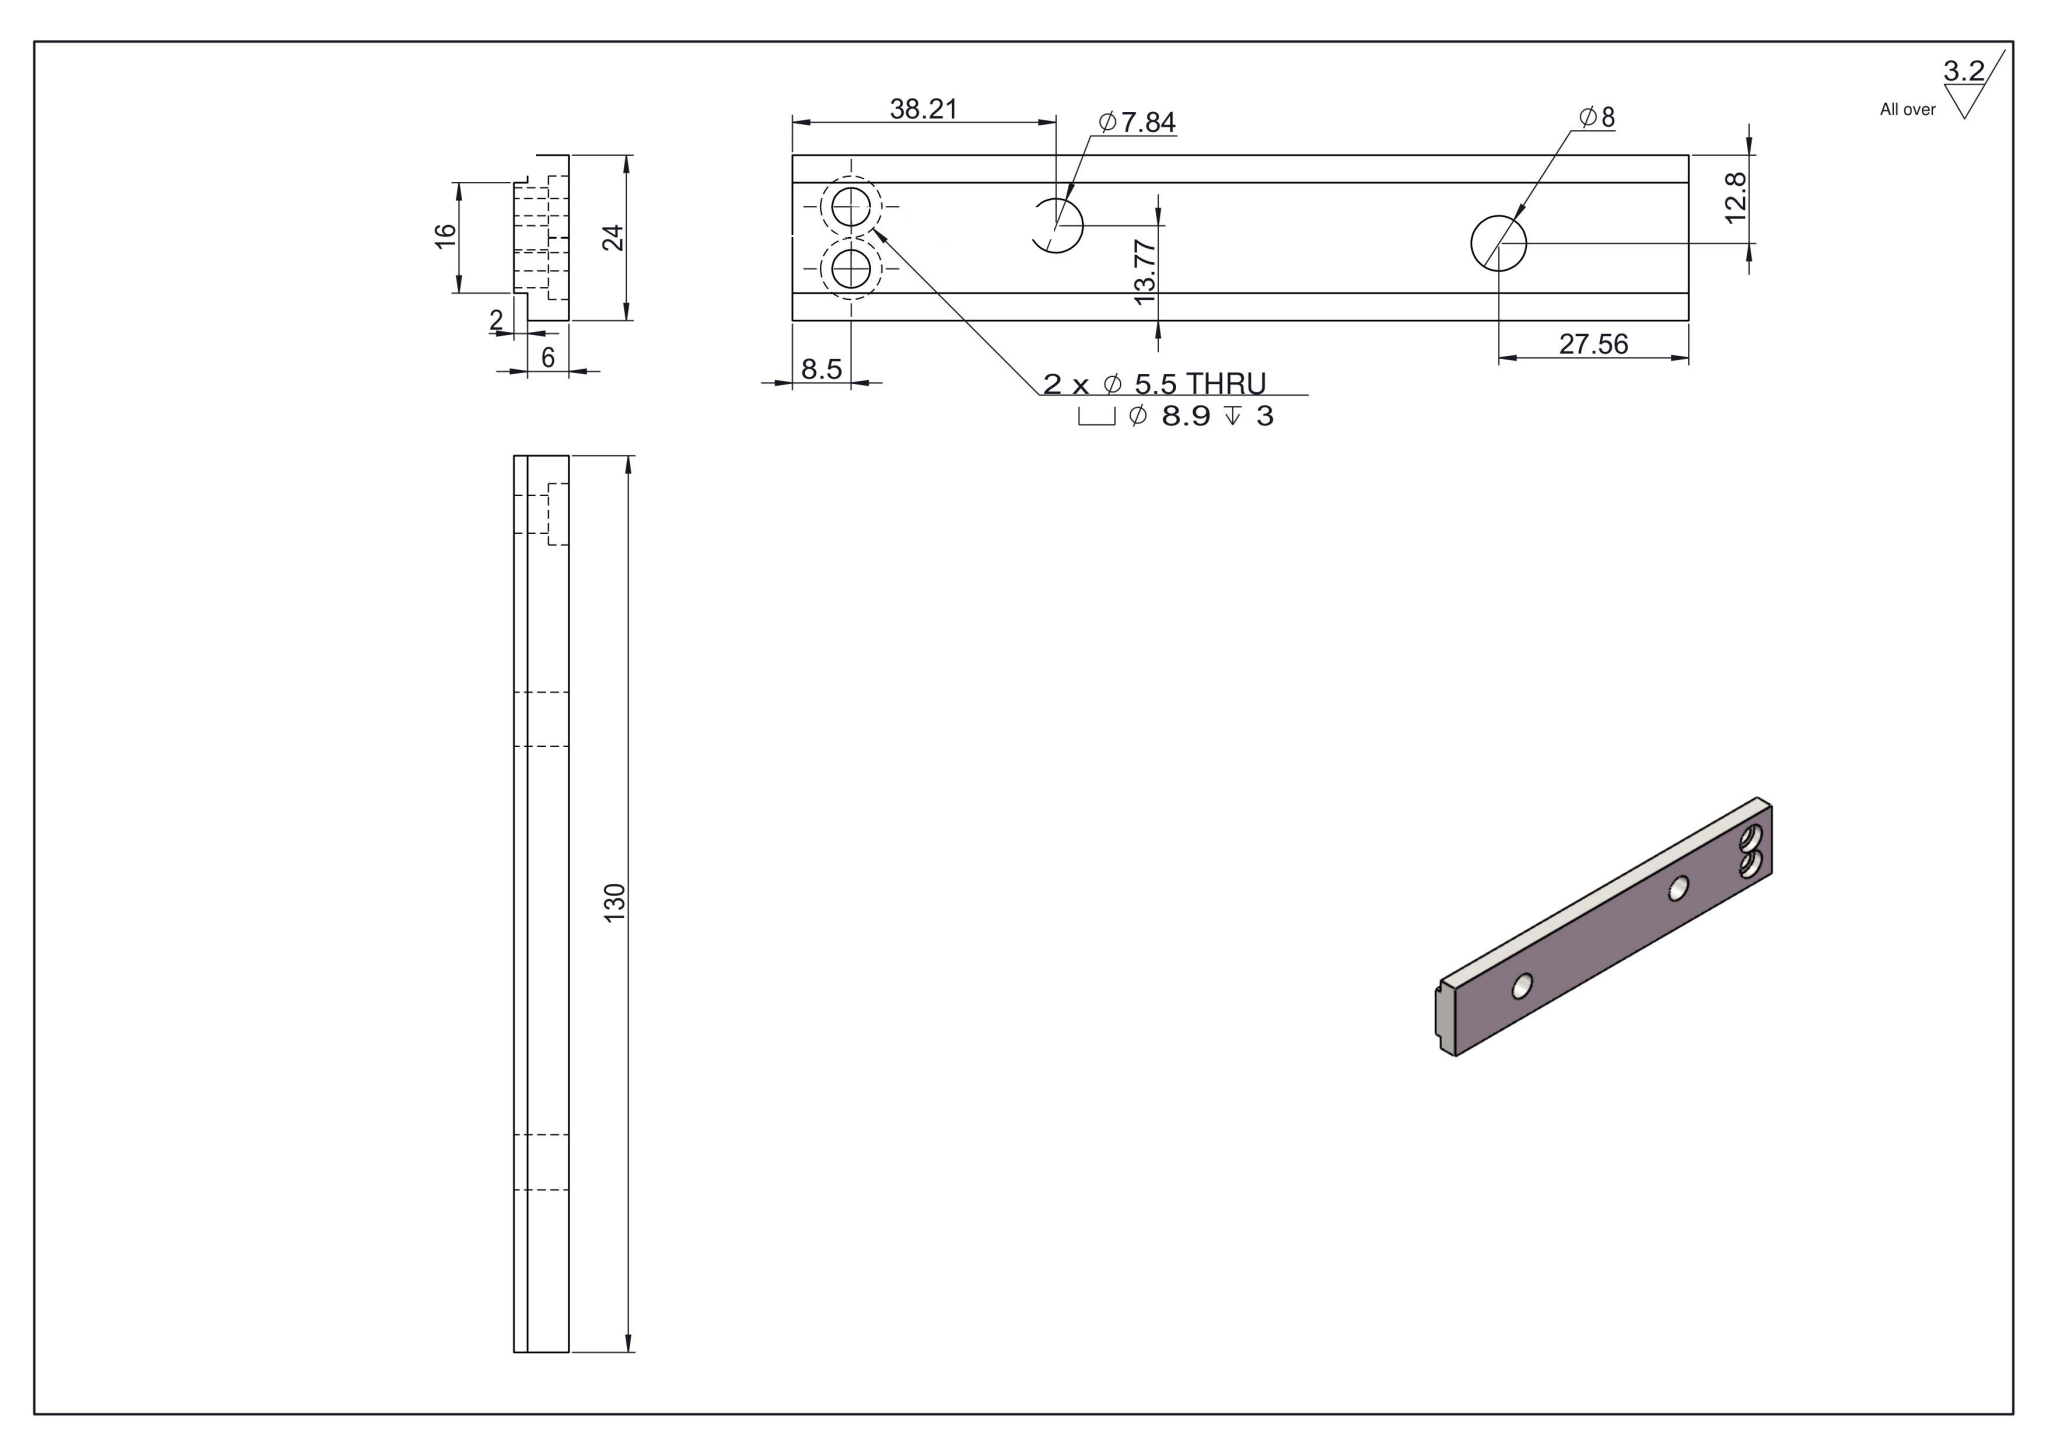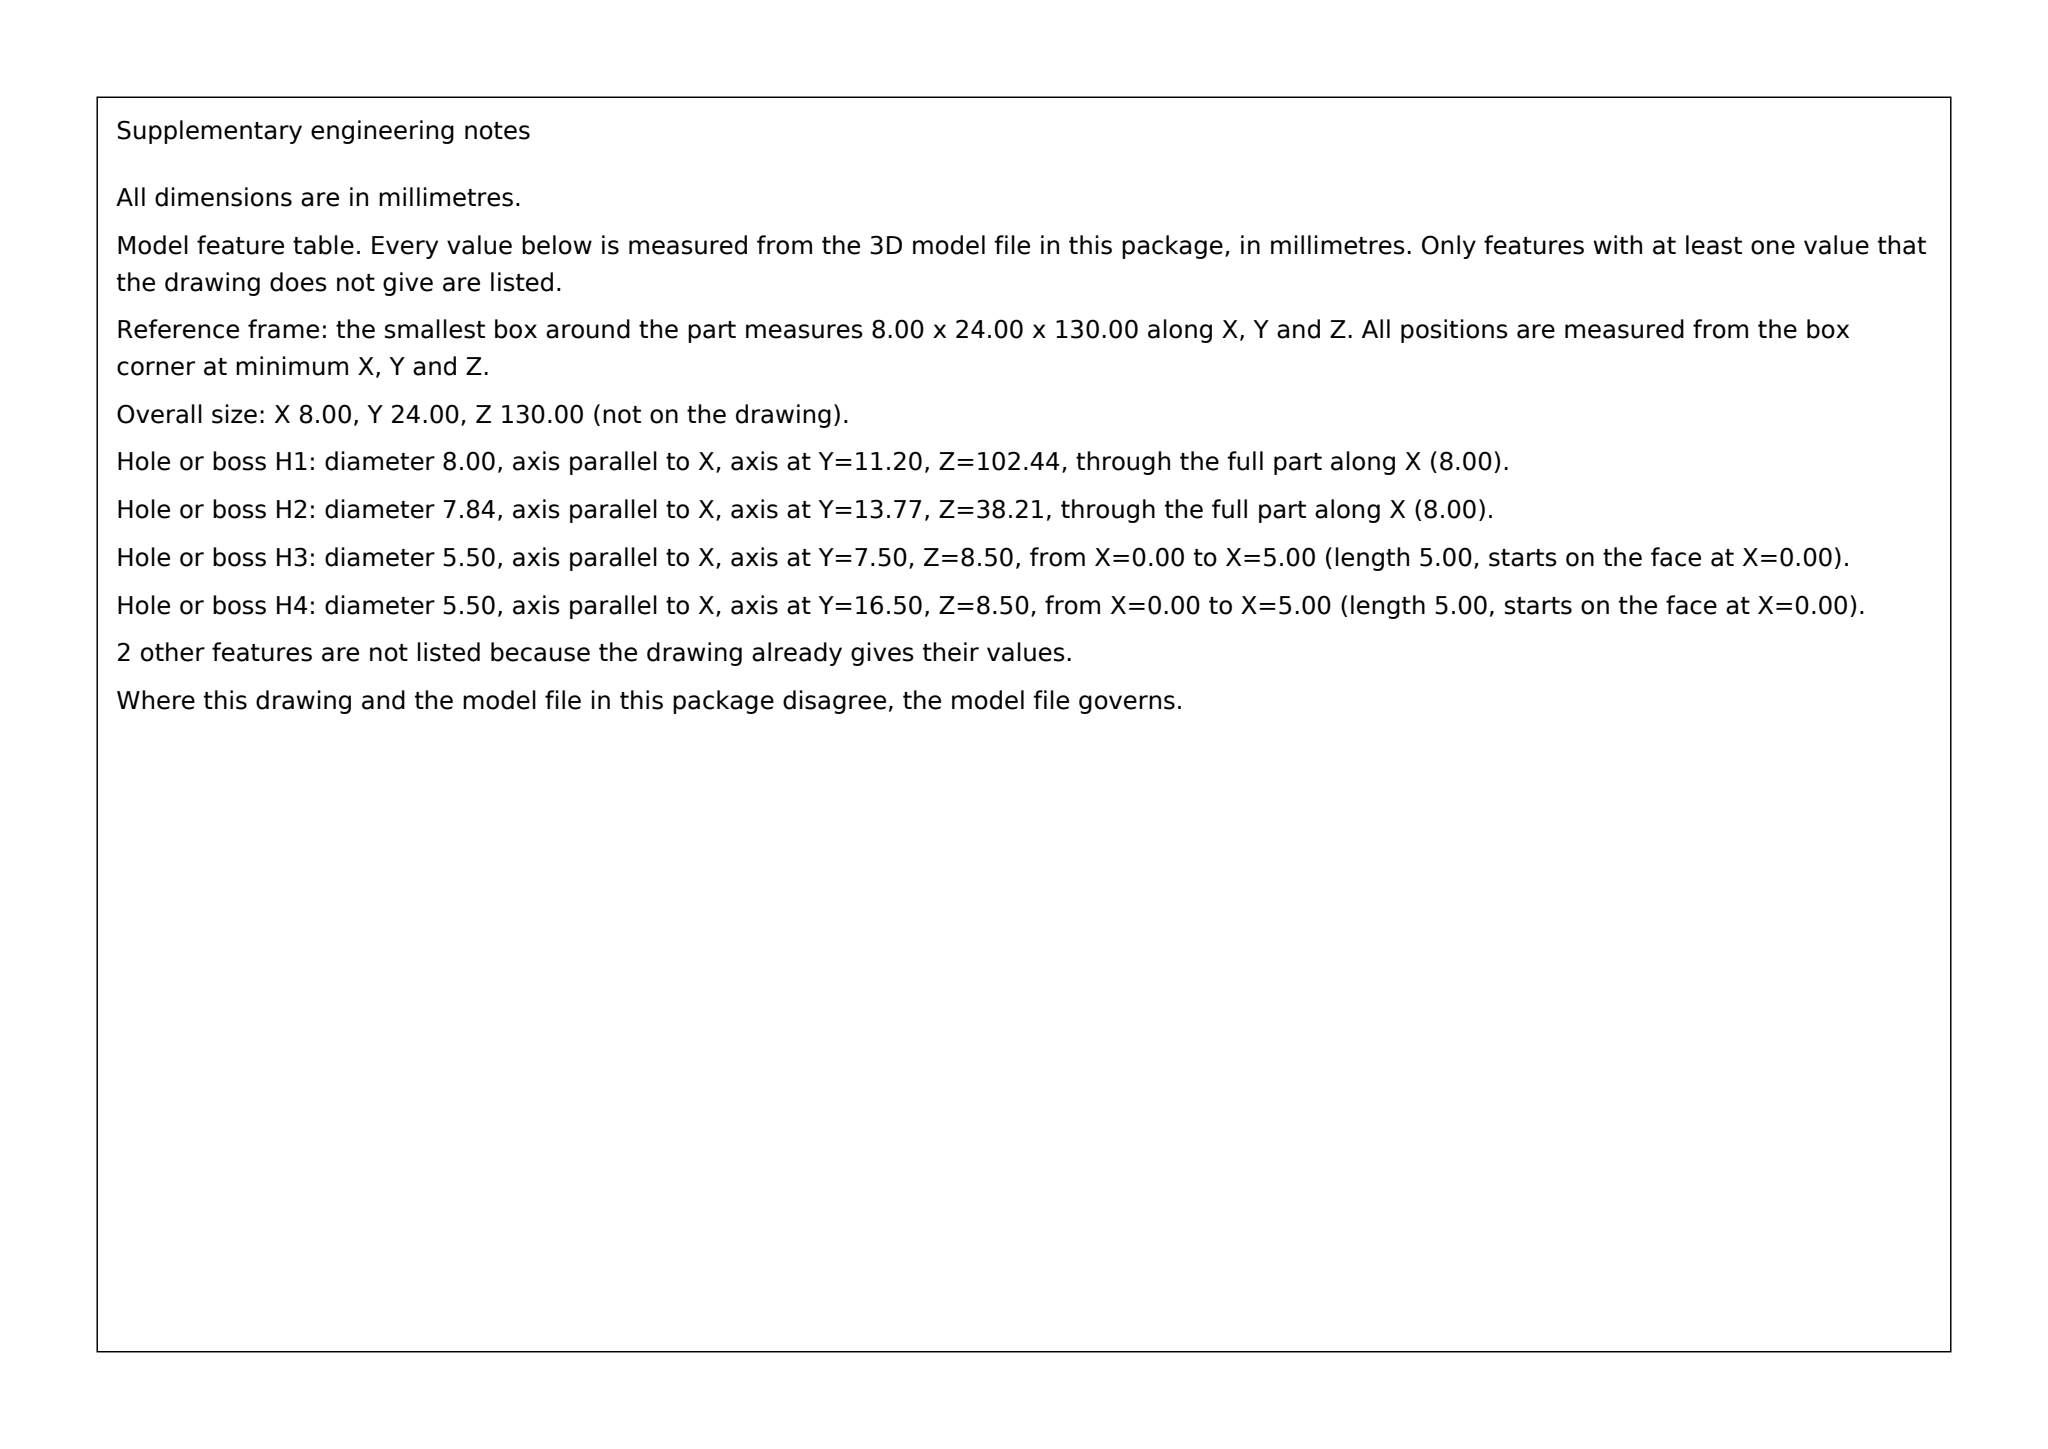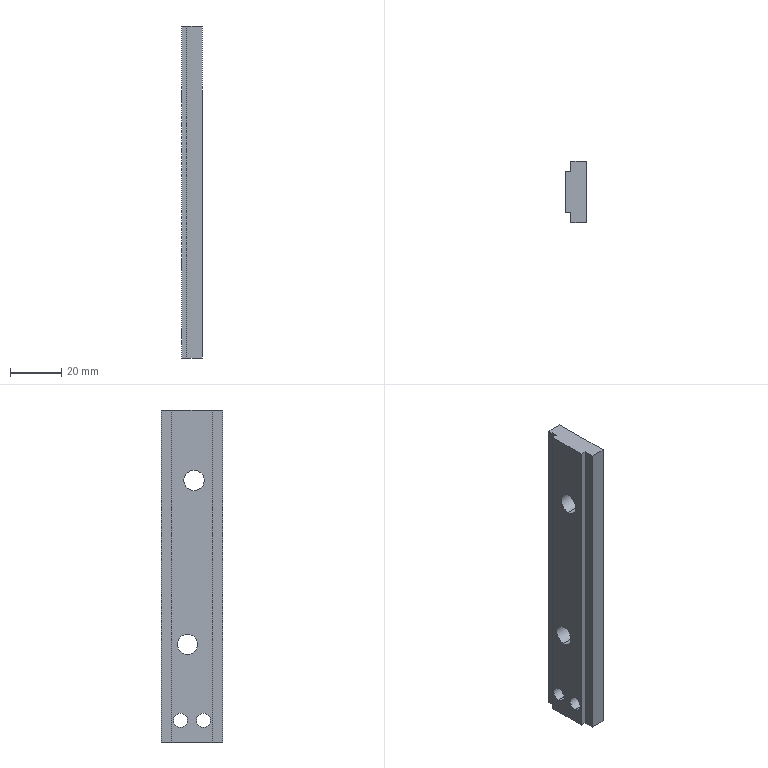Part | SolidWorks | mm | 1 solid | 24 faces | box 8 x 24 x 130 mm | volume 21481 mm3 | cylinder 12 | plane 12 | commonest cylinder face diameters 8.9 x4 5.5 x4 7.84 x2 7.997 x2
build123d program:
from build123d import *

# Parameters (mm, degrees)
BOSS_EXTRUDE1_DEPTH                             = 130
M5_HEX_SOCKET_HEAD_CAP_SCREW_CBORE2_D           = 5.5
M5_HEX_SOCKET_HEAD_CAP_SCREW_CBORE2_CBORE_D     = 8.9
M5_HEX_SOCKET_HEAD_CAP_SCREW_CBORE2_CBORE_DEPTH = 3
SKETCH4_R                                       = 3.92
SKETCH4_R_2                                     = 3.999
CUT_EXTRUDE1_DEPTH                              = 80


with BuildPart() as part:
    # Sketch1 → Boss-Extrude1 (new body)
    with BuildSketch(Plane.XY):
        Polygon((0, 0), (0, -16), (2, -16), (2, -20), (8, -20), (8, 4), (2, 4), (2, 0), align=None)
    extrude(amount=BOSS_EXTRUDE1_DEPTH)

    # M5 Hex Socket Head Cap Screw CBORE2 (through all)
    with Locations(Plane(origin=(8, 0, 0), x_dir=(0, 0, -1), z_dir=(1, 0, 0))):
        with Locations((-8.5, -3.5), (-8.5, -12.5)):
            CounterBoreHole(M5_HEX_SOCKET_HEAD_CAP_SCREW_CBORE2_D / 2, M5_HEX_SOCKET_HEAD_CAP_SCREW_CBORE2_CBORE_D / 2, M5_HEX_SOCKET_HEAD_CAP_SCREW_CBORE2_CBORE_DEPTH)

    # Sketch4 → Cut-Extrude1 (cut)
    with BuildSketch(Plane.ZY):
        with Locations((38.212, -6.229)):
            Circle(SKETCH4_R)
        with Locations((102.442, -8.805)):
            Circle(SKETCH4_R_2)
    extrude(amount=-CUT_EXTRUDE1_DEPTH, mode=Mode.SUBTRACT)


solid = part.part
STEP:
#1=CARTESIAN_POINT('',(8.,-6.229,34.292));
#2=VERTEX_POINT('',#1);
#3=CARTESIAN_POINT('',(8.,-6.229,42.132));
#4=VERTEX_POINT('',#3);
#5=CARTESIAN_POINT('',(8.,-6.229,38.212));
#6=DIRECTION('',(-1.,0.,0.));
#7=DIRECTION('',(0.,0.,1.));
#8=AXIS2_PLACEMENT_3D('',#5,#6,#7);
#9=CIRCLE('',#8,3.92);
#10=EDGE_CURVE('',#2,#4,#9,.T.);
#11=ORIENTED_EDGE('',*,*,#10,.F.);
#12=CARTESIAN_POINT('',(0.,-6.229,34.292));
#13=VERTEX_POINT('',#12);
#14=CARTESIAN_POINT('',(80.,-6.229,34.292));
#15=DIRECTION('',(-1.,0.,0.));
#16=VECTOR('',#15,1000.);
#17=LINE('',#14,#16);
#18=EDGE_CURVE('',#2,#13,#17,.T.);
#19=ORIENTED_EDGE('',*,*,#18,.T.);
#20=CARTESIAN_POINT('',(0.,-6.229,42.132));
#21=VERTEX_POINT('',#20);
#22=CARTESIAN_POINT('',(0.,-6.229,38.212));
#23=DIRECTION('',(-1.,0.,0.));
#24=DIRECTION('',(0.,0.,1.));
#25=AXIS2_PLACEMENT_3D('',#22,#23,#24);
#26=CIRCLE('',#25,3.92);
#27=EDGE_CURVE('',#13,#21,#26,.T.);
#28=ORIENTED_EDGE('',*,*,#27,.T.);
#29=CARTESIAN_POINT('',(80.,-6.229,42.132));
#30=DIRECTION('',(-1.,0.,0.));
#31=VECTOR('',#30,1000.);
#32=LINE('',#29,#31);
#33=EDGE_CURVE('',#4,#21,#32,.T.);
#34=ORIENTED_EDGE('',*,*,#33,.F.);
#35=EDGE_LOOP('',(#11,#19,#28,#34));
#36=FACE_OUTER_BOUND('',#35,.T.);
#37=CARTESIAN_POINT('',(80.,-6.229,38.212));
#38=DIRECTION('',(-1.,0.,0.));
#39=DIRECTION('',(0.,0.,1.));
#40=AXIS2_PLACEMENT_3D('',#37,#38,#39);
#41=CYLINDRICAL_SURFACE('',#40,3.92);
#42=ADVANCED_FACE('',(#36),#41,.F.);
#43=CARTESIAN_POINT('',(8.,-8.805,98.443));
#44=VERTEX_POINT('',#43);
#45=CARTESIAN_POINT('',(8.,-8.805,106.441));
#46=VERTEX_POINT('',#45);
#47=CARTESIAN_POINT('',(8.,-8.805,102.442));
#48=DIRECTION('',(-1.,0.,0.));
#49=DIRECTION('',(0.,0.,1.));
#50=AXIS2_PLACEMENT_3D('',#47,#48,#49);
#51=CIRCLE('',#50,3.999);
#52=EDGE_CURVE('',#44,#46,#51,.T.);
#53=ORIENTED_EDGE('',*,*,#52,.F.);
#54=CARTESIAN_POINT('',(0.,-8.805,98.443));
#55=VERTEX_POINT('',#54);
#56=CARTESIAN_POINT('',(80.,-8.805,98.443));
#57=DIRECTION('',(-1.,0.,0.));
#58=VECTOR('',#57,1000.);
#59=LINE('',#56,#58);
#60=EDGE_CURVE('',#44,#55,#59,.T.);
#61=ORIENTED_EDGE('',*,*,#60,.T.);
#62=CARTESIAN_POINT('',(0.,-8.805,106.441));
#63=VERTEX_POINT('',#62);
#64=CARTESIAN_POINT('',(0.,-8.805,102.442));
#65=DIRECTION('',(-1.,0.,0.));
#66=DIRECTION('',(0.,0.,1.));
#67=AXIS2_PLACEMENT_3D('',#64,#65,#66);
#68=CIRCLE('',#67,3.999);
#69=EDGE_CURVE('',#55,#63,#68,.T.);
#70=ORIENTED_EDGE('',*,*,#69,.T.);
#71=CARTESIAN_POINT('',(80.,-8.805,106.441));
#72=DIRECTION('',(-1.,0.,0.));
#73=VECTOR('',#72,1000.);
#74=LINE('',#71,#73);
#75=EDGE_CURVE('',#46,#63,#74,.T.);
#76=ORIENTED_EDGE('',*,*,#75,.F.);
#77=EDGE_LOOP('',(#53,#61,#70,#76));
#78=FACE_OUTER_BOUND('',#77,.T.);
#79=CARTESIAN_POINT('',(80.,-8.805,102.442));
#80=DIRECTION('',(-1.,0.,0.));
#81=DIRECTION('',(0.,0.,1.));
#82=AXIS2_PLACEMENT_3D('',#79,#80,#81);
#83=CYLINDRICAL_SURFACE('',#82,3.999);
#84=ADVANCED_FACE('',(#78),#83,.F.);
#85=CARTESIAN_POINT('',(5.,-3.5,12.95));
#86=VERTEX_POINT('',#85);
#87=CARTESIAN_POINT('',(5.,-3.5,4.05));
#88=VERTEX_POINT('',#87);
#89=CARTESIAN_POINT('',(5.,-3.5,8.5));
#90=DIRECTION('',(1.,0.,0.));
#91=DIRECTION('',(0.,0.,-1.));
#92=AXIS2_PLACEMENT_3D('',#89,#90,#91);
#93=CIRCLE('',#92,4.45);
#94=EDGE_CURVE('',#86,#88,#93,.T.);
#95=ORIENTED_EDGE('',*,*,#94,.F.);
#96=CARTESIAN_POINT('',(8.,-3.5,12.95));
#97=VERTEX_POINT('',#96);
#98=CARTESIAN_POINT('',(8.,-3.5,12.95));
#99=DIRECTION('',(1.,0.,0.));
#100=VECTOR('',#99,1000.);
#101=LINE('',#98,#100);
#102=EDGE_CURVE('',#86,#97,#101,.T.);
#103=ORIENTED_EDGE('',*,*,#102,.T.);
#104=CARTESIAN_POINT('',(8.,-3.5,4.05));
#105=VERTEX_POINT('',#104);
#106=CARTESIAN_POINT('',(8.,-3.5,8.5));
#107=DIRECTION('',(1.,0.,0.));
#108=DIRECTION('',(0.,0.,-1.));
#109=AXIS2_PLACEMENT_3D('',#106,#107,#108);
#110=CIRCLE('',#109,4.45);
#111=EDGE_CURVE('',#97,#105,#110,.T.);
#112=ORIENTED_EDGE('',*,*,#111,.T.);
#113=CARTESIAN_POINT('',(8.,-3.5,4.05));
#114=DIRECTION('',(1.,0.,0.));
#115=VECTOR('',#114,1000.);
#116=LINE('',#113,#115);
#117=EDGE_CURVE('',#88,#105,#116,.T.);
#118=ORIENTED_EDGE('',*,*,#117,.F.);
#119=EDGE_LOOP('',(#95,#103,#112,#118));
#120=FACE_OUTER_BOUND('',#119,.T.);
#121=CARTESIAN_POINT('',(8.,-3.5,8.5));
#122=DIRECTION('',(1.,0.,0.));
#123=DIRECTION('',(0.,0.,-1.));
#124=AXIS2_PLACEMENT_3D('',#121,#122,#123);
#125=CYLINDRICAL_SURFACE('',#124,4.45);
#126=ADVANCED_FACE('',(#120),#125,.F.);
#127=CARTESIAN_POINT('',(0.,-3.5,11.25));
#128=VERTEX_POINT('',#127);
#129=CARTESIAN_POINT('',(0.,-3.5,5.75));
#130=VERTEX_POINT('',#129);
#131=CARTESIAN_POINT('',(0.,-3.5,8.5));
#132=DIRECTION('',(1.,0.,0.));
#133=DIRECTION('',(0.,0.,-1.));
#134=AXIS2_PLACEMENT_3D('',#131,#132,#133);
#135=CIRCLE('',#134,2.75);
#136=EDGE_CURVE('',#128,#130,#135,.T.);
#137=ORIENTED_EDGE('',*,*,#136,.F.);
#138=CARTESIAN_POINT('',(5.,-3.5,11.25));
#139=VERTEX_POINT('',#138);
#140=CARTESIAN_POINT('',(8.,-3.5,11.25));
#141=DIRECTION('',(1.,0.,0.));
#142=VECTOR('',#141,1000.);
#143=LINE('',#140,#142);
#144=EDGE_CURVE('',#128,#139,#143,.T.);
#145=ORIENTED_EDGE('',*,*,#144,.T.);
#146=CARTESIAN_POINT('',(5.,-3.5,5.75));
#147=VERTEX_POINT('',#146);
#148=CARTESIAN_POINT('',(5.,-3.5,8.5));
#149=DIRECTION('',(1.,0.,0.));
#150=DIRECTION('',(0.,0.,-1.));
#151=AXIS2_PLACEMENT_3D('',#148,#149,#150);
#152=CIRCLE('',#151,2.75);
#153=EDGE_CURVE('',#139,#147,#152,.T.);
#154=ORIENTED_EDGE('',*,*,#153,.T.);
#155=CARTESIAN_POINT('',(8.,-3.5,5.75));
#156=DIRECTION('',(1.,0.,0.));
#157=VECTOR('',#156,1000.);
#158=LINE('',#155,#157);
#159=EDGE_CURVE('',#130,#147,#158,.T.);
#160=ORIENTED_EDGE('',*,*,#159,.F.);
#161=EDGE_LOOP('',(#137,#145,#154,#160));
#162=FACE_OUTER_BOUND('',#161,.T.);
#163=CARTESIAN_POINT('',(8.,-3.5,8.5));
#164=DIRECTION('',(1.,0.,0.));
#165=DIRECTION('',(0.,0.,-1.));
#166=AXIS2_PLACEMENT_3D('',#163,#164,#165);
#167=CYLINDRICAL_SURFACE('',#166,2.75);
#168=ADVANCED_FACE('',(#162),#167,.F.);
#169=CARTESIAN_POINT('',(5.,-12.5,12.95));
#170=VERTEX_POINT('',#169);
#171=CARTESIAN_POINT('',(5.,-12.5,4.05));
#172=VERTEX_POINT('',#171);
#173=CARTESIAN_POINT('',(5.,-12.5,8.5));
#174=DIRECTION('',(1.,0.,0.));
#175=DIRECTION('',(0.,0.,-1.));
#176=AXIS2_PLACEMENT_3D('',#173,#174,#175);
#177=CIRCLE('',#176,4.45);
#178=EDGE_CURVE('',#170,#172,#177,.T.);
#179=ORIENTED_EDGE('',*,*,#178,.F.);
#180=CARTESIAN_POINT('',(8.,-12.5,12.95));
#181=VERTEX_POINT('',#180);
#182=CARTESIAN_POINT('',(8.,-12.5,12.95));
#183=DIRECTION('',(1.,0.,0.));
#184=VECTOR('',#183,1000.);
#185=LINE('',#182,#184);
#186=EDGE_CURVE('',#170,#181,#185,.T.);
#187=ORIENTED_EDGE('',*,*,#186,.T.);
#188=CARTESIAN_POINT('',(8.,-12.5,4.05));
#189=VERTEX_POINT('',#188);
#190=CARTESIAN_POINT('',(8.,-12.5,8.5));
#191=DIRECTION('',(1.,0.,0.));
#192=DIRECTION('',(0.,0.,-1.));
#193=AXIS2_PLACEMENT_3D('',#190,#191,#192);
#194=CIRCLE('',#193,4.45);
#195=EDGE_CURVE('',#181,#189,#194,.T.);
#196=ORIENTED_EDGE('',*,*,#195,.T.);
#197=CARTESIAN_POINT('',(8.,-12.5,4.05));
#198=DIRECTION('',(1.,0.,0.));
#199=VECTOR('',#198,1000.);
#200=LINE('',#197,#199);
#201=EDGE_CURVE('',#172,#189,#200,.T.);
#202=ORIENTED_EDGE('',*,*,#201,.F.);
#203=EDGE_LOOP('',(#179,#187,#196,#202));
#204=FACE_OUTER_BOUND('',#203,.T.);
#205=CARTESIAN_POINT('',(8.,-12.5,8.5));
#206=DIRECTION('',(1.,0.,0.));
#207=DIRECTION('',(0.,0.,-1.));
#208=AXIS2_PLACEMENT_3D('',#205,#206,#207);
#209=CYLINDRICAL_SURFACE('',#208,4.45);
#210=ADVANCED_FACE('',(#204),#209,.F.);
#211=CARTESIAN_POINT('',(0.,-12.5,11.25));
#212=VERTEX_POINT('',#211);
#213=CARTESIAN_POINT('',(0.,-12.5,5.75));
#214=VERTEX_POINT('',#213);
#215=CARTESIAN_POINT('',(0.,-12.5,8.5));
#216=DIRECTION('',(1.,0.,0.));
#217=DIRECTION('',(0.,0.,-1.));
#218=AXIS2_PLACEMENT_3D('',#215,#216,#217);
#219=CIRCLE('',#218,2.75);
#220=EDGE_CURVE('',#212,#214,#219,.T.);
#221=ORIENTED_EDGE('',*,*,#220,.F.);
#222=CARTESIAN_POINT('',(5.,-12.5,11.25));
#223=VERTEX_POINT('',#222);
#224=CARTESIAN_POINT('',(8.,-12.5,11.25));
#225=DIRECTION('',(1.,0.,0.));
#226=VECTOR('',#225,1000.);
#227=LINE('',#224,#226);
#228=EDGE_CURVE('',#212,#223,#227,.T.);
#229=ORIENTED_EDGE('',*,*,#228,.T.);
#230=CARTESIAN_POINT('',(5.,-12.5,5.75));
#231=VERTEX_POINT('',#230);
#232=CARTESIAN_POINT('',(5.,-12.5,8.5));
#233=DIRECTION('',(1.,0.,0.));
#234=DIRECTION('',(0.,0.,-1.));
#235=AXIS2_PLACEMENT_3D('',#232,#233,#234);
#236=CIRCLE('',#235,2.75);
#237=EDGE_CURVE('',#223,#231,#236,.T.);
#238=ORIENTED_EDGE('',*,*,#237,.T.);
#239=CARTESIAN_POINT('',(8.,-12.5,5.75));
#240=DIRECTION('',(1.,0.,0.));
#241=VECTOR('',#240,1000.);
#242=LINE('',#239,#241);
#243=EDGE_CURVE('',#214,#231,#242,.T.);
#244=ORIENTED_EDGE('',*,*,#243,.F.);
#245=EDGE_LOOP('',(#221,#229,#238,#244));
#246=FACE_OUTER_BOUND('',#245,.T.);
#247=CARTESIAN_POINT('',(8.,-12.5,8.5));
#248=DIRECTION('',(1.,0.,0.));
#249=DIRECTION('',(0.,0.,-1.));
#250=AXIS2_PLACEMENT_3D('',#247,#248,#249);
#251=CYLINDRICAL_SURFACE('',#250,2.75);
#252=ADVANCED_FACE('',(#246),#251,.F.);
#253=CARTESIAN_POINT('',(8.,-6.229,38.212));
#254=DIRECTION('',(-1.,0.,0.));
#255=DIRECTION('',(0.,0.,1.));
#256=AXIS2_PLACEMENT_3D('',#253,#254,#255);
#257=CIRCLE('',#256,3.92);
#258=EDGE_CURVE('',#4,#2,#257,.T.);
#259=ORIENTED_EDGE('',*,*,#258,.T.);
#260=ORIENTED_EDGE('',*,*,#10,.T.);
#261=EDGE_LOOP('',(#259,#260));
#262=FACE_BOUND('',#261,.T.);
#263=CARTESIAN_POINT('',(8.,-8.805,102.442));
#264=DIRECTION('',(-1.,0.,0.));
#265=DIRECTION('',(0.,0.,1.));
#266=AXIS2_PLACEMENT_3D('',#263,#264,#265);
#267=CIRCLE('',#266,3.999);
#268=EDGE_CURVE('',#46,#44,#267,.T.);
#269=ORIENTED_EDGE('',*,*,#268,.T.);
#270=ORIENTED_EDGE('',*,*,#52,.T.);
#271=EDGE_LOOP('',(#269,#270));
#272=FACE_BOUND('',#271,.T.);
#273=CARTESIAN_POINT('',(8.,-12.5,8.5));
#274=DIRECTION('',(1.,0.,0.));
#275=DIRECTION('',(0.,0.,-1.));
#276=AXIS2_PLACEMENT_3D('',#273,#274,#275);
#277=CIRCLE('',#276,4.45);
#278=EDGE_CURVE('',#189,#181,#277,.T.);
#279=ORIENTED_EDGE('',*,*,#278,.F.);
#280=ORIENTED_EDGE('',*,*,#195,.F.);
#281=EDGE_LOOP('',(#279,#280));
#282=FACE_BOUND('',#281,.T.);
#283=CARTESIAN_POINT('',(8.,-20.,0.));
#284=VERTEX_POINT('',#283);
#285=CARTESIAN_POINT('',(8.,4.,0.));
#286=VERTEX_POINT('',#285);
#287=CARTESIAN_POINT('',(8.,-20.,0.));
#288=DIRECTION('',(0.,1.,0.));
#289=VECTOR('',#288,1000.);
#290=LINE('',#287,#289);
#291=EDGE_CURVE('',#284,#286,#290,.T.);
#292=ORIENTED_EDGE('',*,*,#291,.T.);
#293=CARTESIAN_POINT('',(8.,4.,130.));
#294=VERTEX_POINT('',#293);
#295=CARTESIAN_POINT('',(8.,4.,130.));
#296=DIRECTION('',(0.,0.,-1.));
#297=VECTOR('',#296,1000.);
#298=LINE('',#295,#297);
#299=EDGE_CURVE('',#294,#286,#298,.T.);
#300=ORIENTED_EDGE('',*,*,#299,.F.);
#301=CARTESIAN_POINT('',(8.,-20.,130.));
#302=VERTEX_POINT('',#301);
#303=CARTESIAN_POINT('',(8.,-20.,130.));
#304=DIRECTION('',(0.,1.,0.));
#305=VECTOR('',#304,1000.);
#306=LINE('',#303,#305);
#307=EDGE_CURVE('',#302,#294,#306,.T.);
#308=ORIENTED_EDGE('',*,*,#307,.F.);
#309=CARTESIAN_POINT('',(8.,-20.,130.));
#310=DIRECTION('',(0.,0.,-1.));
#311=VECTOR('',#310,1000.);
#312=LINE('',#309,#311);
#313=EDGE_CURVE('',#302,#284,#312,.T.);
#314=ORIENTED_EDGE('',*,*,#313,.T.);
#315=EDGE_LOOP('',(#292,#300,#308,#314));
#316=FACE_OUTER_BOUND('',#315,.T.);
#317=CARTESIAN_POINT('',(8.,-3.5,8.5));
#318=DIRECTION('',(1.,0.,0.));
#319=DIRECTION('',(0.,0.,-1.));
#320=AXIS2_PLACEMENT_3D('',#317,#318,#319);
#321=CIRCLE('',#320,4.45);
#322=EDGE_CURVE('',#105,#97,#321,.T.);
#323=ORIENTED_EDGE('',*,*,#322,.F.);
#324=ORIENTED_EDGE('',*,*,#111,.F.);
#325=EDGE_LOOP('',(#323,#324));
#326=FACE_BOUND('',#325,.T.);
#327=CARTESIAN_POINT('',(8.,-20.,130.));
#328=DIRECTION('',(-1.,0.,0.));
#329=DIRECTION('',(0.,0.,1.));
#330=AXIS2_PLACEMENT_3D('',#327,#328,#329);
#331=PLANE('',#330);
#332=ADVANCED_FACE('',(#262,#272,#282,#316,#326),#331,.F.);
#333=CARTESIAN_POINT('',(2.,-0.,0.));
#334=VERTEX_POINT('',#333);
#335=CARTESIAN_POINT('',(0.,0.,0.));
#336=VERTEX_POINT('',#335);
#337=CARTESIAN_POINT('',(2.,-0.,0.));
#338=DIRECTION('',(-1.,0.,0.));
#339=VECTOR('',#338,1000.);
#340=LINE('',#337,#339);
#341=EDGE_CURVE('',#334,#336,#340,.T.);
#342=ORIENTED_EDGE('',*,*,#341,.T.);
#343=CARTESIAN_POINT('',(0.,0.,130.));
#344=VERTEX_POINT('',#343);
#345=CARTESIAN_POINT('',(0.,0.,130.));
#346=DIRECTION('',(0.,0.,-1.));
#347=VECTOR('',#346,1000.);
#348=LINE('',#345,#347);
#349=EDGE_CURVE('',#344,#336,#348,.T.);
#350=ORIENTED_EDGE('',*,*,#349,.F.);
#351=CARTESIAN_POINT('',(2.,-0.,130.));
#352=VERTEX_POINT('',#351);
#353=CARTESIAN_POINT('',(2.,-0.,130.));
#354=DIRECTION('',(-1.,0.,0.));
#355=VECTOR('',#354,1000.);
#356=LINE('',#353,#355);
#357=EDGE_CURVE('',#352,#344,#356,.T.);
#358=ORIENTED_EDGE('',*,*,#357,.F.);
#359=CARTESIAN_POINT('',(2.,-0.,130.));
#360=DIRECTION('',(0.,0.,-1.));
#361=VECTOR('',#360,1000.);
#362=LINE('',#359,#361);
#363=EDGE_CURVE('',#352,#334,#362,.T.);
#364=ORIENTED_EDGE('',*,*,#363,.T.);
#365=EDGE_LOOP('',(#342,#350,#358,#364));
#366=FACE_OUTER_BOUND('',#365,.T.);
#367=CARTESIAN_POINT('',(2.,-0.,130.));
#368=DIRECTION('',(-0.,-1.,0.));
#369=DIRECTION('',(1.,-0.,0.));
#370=AXIS2_PLACEMENT_3D('',#367,#368,#369);
#371=PLANE('',#370);
#372=ADVANCED_FACE('',(#366),#371,.F.);
#373=CARTESIAN_POINT('',(0.,-6.229,38.212));
#374=DIRECTION('',(-1.,0.,0.));
#375=DIRECTION('',(0.,0.,1.));
#376=AXIS2_PLACEMENT_3D('',#373,#374,#375);
#377=CIRCLE('',#376,3.92);
#378=EDGE_CURVE('',#21,#13,#377,.T.);
#379=ORIENTED_EDGE('',*,*,#378,.F.);
#380=ORIENTED_EDGE('',*,*,#27,.F.);
#381=EDGE_LOOP('',(#379,#380));
#382=FACE_BOUND('',#381,.T.);
#383=CARTESIAN_POINT('',(0.,-8.805,102.442));
#384=DIRECTION('',(-1.,0.,0.));
#385=DIRECTION('',(0.,0.,1.));
#386=AXIS2_PLACEMENT_3D('',#383,#384,#385);
#387=CIRCLE('',#386,3.999);
#388=EDGE_CURVE('',#63,#55,#387,.T.);
#389=ORIENTED_EDGE('',*,*,#388,.F.);
#390=ORIENTED_EDGE('',*,*,#69,.F.);
#391=EDGE_LOOP('',(#389,#390));
#392=FACE_BOUND('',#391,.T.);
#393=CARTESIAN_POINT('',(0.,-3.5,8.5));
#394=DIRECTION('',(1.,0.,0.));
#395=DIRECTION('',(0.,0.,-1.));
#396=AXIS2_PLACEMENT_3D('',#393,#394,#395);
#397=CIRCLE('',#396,2.75);
#398=EDGE_CURVE('',#130,#128,#397,.T.);
#399=ORIENTED_EDGE('',*,*,#398,.T.);
#400=ORIENTED_EDGE('',*,*,#136,.T.);
#401=EDGE_LOOP('',(#399,#400));
#402=FACE_BOUND('',#401,.T.);
#403=CARTESIAN_POINT('',(0.,-12.5,8.5));
#404=DIRECTION('',(1.,0.,0.));
#405=DIRECTION('',(0.,0.,-1.));
#406=AXIS2_PLACEMENT_3D('',#403,#404,#405);
#407=CIRCLE('',#406,2.75);
#408=EDGE_CURVE('',#214,#212,#407,.T.);
#409=ORIENTED_EDGE('',*,*,#408,.T.);
#410=ORIENTED_EDGE('',*,*,#220,.T.);
#411=EDGE_LOOP('',(#409,#410));
#412=FACE_BOUND('',#411,.T.);
#413=CARTESIAN_POINT('',(0.,-16.,0.));
#414=VERTEX_POINT('',#413);
#415=CARTESIAN_POINT('',(0.,0.,0.));
#416=DIRECTION('',(0.,-1.,0.));
#417=VECTOR('',#416,1000.);
#418=LINE('',#415,#417);
#419=EDGE_CURVE('',#336,#414,#418,.T.);
#420=ORIENTED_EDGE('',*,*,#419,.T.);
#421=CARTESIAN_POINT('',(0.,-16.,130.));
#422=VERTEX_POINT('',#421);
#423=CARTESIAN_POINT('',(0.,-16.,130.));
#424=DIRECTION('',(0.,0.,-1.));
#425=VECTOR('',#424,1000.);
#426=LINE('',#423,#425);
#427=EDGE_CURVE('',#422,#414,#426,.T.);
#428=ORIENTED_EDGE('',*,*,#427,.F.);
#429=CARTESIAN_POINT('',(0.,0.,130.));
#430=DIRECTION('',(0.,-1.,0.));
#431=VECTOR('',#430,1000.);
#432=LINE('',#429,#431);
#433=EDGE_CURVE('',#344,#422,#432,.T.);
#434=ORIENTED_EDGE('',*,*,#433,.F.);
#435=ORIENTED_EDGE('',*,*,#349,.T.);
#436=EDGE_LOOP('',(#420,#428,#434,#435));
#437=FACE_OUTER_BOUND('',#436,.T.);
#438=CARTESIAN_POINT('',(0.,0.,130.));
#439=DIRECTION('',(1.,0.,0.));
#440=DIRECTION('',(0.,0.,-1.));
#441=AXIS2_PLACEMENT_3D('',#438,#439,#440);
#442=PLANE('',#441);
#443=ADVANCED_FACE('',(#382,#392,#402,#412,#437),#442,.F.);
#444=CARTESIAN_POINT('',(2.,-16.,0.));
#445=VERTEX_POINT('',#444);
#446=CARTESIAN_POINT('',(0.,-16.,0.));
#447=DIRECTION('',(1.,0.,0.));
#448=VECTOR('',#447,1000.);
#449=LINE('',#446,#448);
#450=EDGE_CURVE('',#414,#445,#449,.T.);
#451=ORIENTED_EDGE('',*,*,#450,.T.);
#452=CARTESIAN_POINT('',(2.,-16.,130.));
#453=VERTEX_POINT('',#452);
#454=CARTESIAN_POINT('',(2.,-16.,130.));
#455=DIRECTION('',(0.,0.,-1.));
#456=VECTOR('',#455,1000.);
#457=LINE('',#454,#456);
#458=EDGE_CURVE('',#453,#445,#457,.T.);
#459=ORIENTED_EDGE('',*,*,#458,.F.);
#460=CARTESIAN_POINT('',(0.,-16.,130.));
#461=DIRECTION('',(1.,0.,0.));
#462=VECTOR('',#461,1000.);
#463=LINE('',#460,#462);
#464=EDGE_CURVE('',#422,#453,#463,.T.);
#465=ORIENTED_EDGE('',*,*,#464,.F.);
#466=ORIENTED_EDGE('',*,*,#427,.T.);
#467=EDGE_LOOP('',(#451,#459,#465,#466));
#468=FACE_OUTER_BOUND('',#467,.T.);
#469=CARTESIAN_POINT('',(0.,-16.,130.));
#470=DIRECTION('',(0.,1.,0.));
#471=DIRECTION('',(0.,0.,1.));
#472=AXIS2_PLACEMENT_3D('',#469,#470,#471);
#473=PLANE('',#472);
#474=ADVANCED_FACE('',(#468),#473,.F.);
#475=CARTESIAN_POINT('',(2.,-20.,0.));
#476=VERTEX_POINT('',#475);
#477=CARTESIAN_POINT('',(2.,-16.,0.));
#478=DIRECTION('',(0.,-1.,0.));
#479=VECTOR('',#478,1000.);
#480=LINE('',#477,#479);
#481=EDGE_CURVE('',#445,#476,#480,.T.);
#482=ORIENTED_EDGE('',*,*,#481,.T.);
#483=CARTESIAN_POINT('',(2.,-20.,130.));
#484=VERTEX_POINT('',#483);
#485=CARTESIAN_POINT('',(2.,-20.,130.));
#486=DIRECTION('',(0.,0.,-1.));
#487=VECTOR('',#486,1000.);
#488=LINE('',#485,#487);
#489=EDGE_CURVE('',#484,#476,#488,.T.);
#490=ORIENTED_EDGE('',*,*,#489,.F.);
#491=CARTESIAN_POINT('',(2.,-16.,130.));
#492=DIRECTION('',(0.,-1.,0.));
#493=VECTOR('',#492,1000.);
#494=LINE('',#491,#493);
#495=EDGE_CURVE('',#453,#484,#494,.T.);
#496=ORIENTED_EDGE('',*,*,#495,.F.);
#497=ORIENTED_EDGE('',*,*,#458,.T.);
#498=EDGE_LOOP('',(#482,#490,#496,#497));
#499=FACE_OUTER_BOUND('',#498,.T.);
#500=CARTESIAN_POINT('',(2.,-16.,130.));
#501=DIRECTION('',(1.,0.,0.));
#502=DIRECTION('',(0.,0.,-1.));
#503=AXIS2_PLACEMENT_3D('',#500,#501,#502);
#504=PLANE('',#503);
#505=ADVANCED_FACE('',(#499),#504,.F.);
#506=CARTESIAN_POINT('',(2.,-20.,0.));
#507=DIRECTION('',(1.,0.,0.));
#508=VECTOR('',#507,1000.);
#509=LINE('',#506,#508);
#510=EDGE_CURVE('',#476,#284,#509,.T.);
#511=ORIENTED_EDGE('',*,*,#510,.T.);
#512=ORIENTED_EDGE('',*,*,#313,.F.);
#513=CARTESIAN_POINT('',(2.,-20.,130.));
#514=DIRECTION('',(1.,0.,0.));
#515=VECTOR('',#514,1000.);
#516=LINE('',#513,#515);
#517=EDGE_CURVE('',#484,#302,#516,.T.);
#518=ORIENTED_EDGE('',*,*,#517,.F.);
#519=ORIENTED_EDGE('',*,*,#489,.T.);
#520=EDGE_LOOP('',(#511,#512,#518,#519));
#521=FACE_OUTER_BOUND('',#520,.T.);
#522=CARTESIAN_POINT('',(2.,-20.,130.));
#523=DIRECTION('',(0.,1.,0.));
#524=DIRECTION('',(0.,0.,1.));
#525=AXIS2_PLACEMENT_3D('',#522,#523,#524);
#526=PLANE('',#525);
#527=ADVANCED_FACE('',(#521),#526,.F.);
#528=CARTESIAN_POINT('',(2.,4.,0.));
#529=VERTEX_POINT('',#528);
#530=CARTESIAN_POINT('',(8.,4.,0.));
#531=DIRECTION('',(-1.,0.,0.));
#532=VECTOR('',#531,1000.);
#533=LINE('',#530,#532);
#534=EDGE_CURVE('',#286,#529,#533,.T.);
#535=ORIENTED_EDGE('',*,*,#534,.T.);
#536=CARTESIAN_POINT('',(2.,4.,130.));
#537=VERTEX_POINT('',#536);
#538=CARTESIAN_POINT('',(2.,4.,130.));
#539=DIRECTION('',(0.,0.,-1.));
#540=VECTOR('',#539,1000.);
#541=LINE('',#538,#540);
#542=EDGE_CURVE('',#537,#529,#541,.T.);
#543=ORIENTED_EDGE('',*,*,#542,.F.);
#544=CARTESIAN_POINT('',(8.,4.,130.));
#545=DIRECTION('',(-1.,0.,0.));
#546=VECTOR('',#545,1000.);
#547=LINE('',#544,#546);
#548=EDGE_CURVE('',#294,#537,#547,.T.);
#549=ORIENTED_EDGE('',*,*,#548,.F.);
#550=ORIENTED_EDGE('',*,*,#299,.T.);
#551=EDGE_LOOP('',(#535,#543,#549,#550));
#552=FACE_OUTER_BOUND('',#551,.T.);
#553=CARTESIAN_POINT('',(8.,4.,130.));
#554=DIRECTION('',(0.,-1.,0.));
#555=DIRECTION('',(0.,0.,-1.));
#556=AXIS2_PLACEMENT_3D('',#553,#554,#555);
#557=PLANE('',#556);
#558=ADVANCED_FACE('',(#552),#557,.F.);
#559=CARTESIAN_POINT('',(2.,4.,0.));
#560=DIRECTION('',(-0.,-1.,0.));
#561=VECTOR('',#560,1000.);
#562=LINE('',#559,#561);
#563=EDGE_CURVE('',#529,#334,#562,.T.);
#564=ORIENTED_EDGE('',*,*,#563,.T.);
#565=ORIENTED_EDGE('',*,*,#363,.F.);
#566=CARTESIAN_POINT('',(2.,4.,130.));
#567=DIRECTION('',(-0.,-1.,0.));
#568=VECTOR('',#567,1000.);
#569=LINE('',#566,#568);
#570=EDGE_CURVE('',#537,#352,#569,.T.);
#571=ORIENTED_EDGE('',*,*,#570,.F.);
#572=ORIENTED_EDGE('',*,*,#542,.T.);
#573=EDGE_LOOP('',(#564,#565,#571,#572));
#574=FACE_OUTER_BOUND('',#573,.T.);
#575=CARTESIAN_POINT('',(2.,4.,130.));
#576=DIRECTION('',(1.,-0.,0.));
#577=DIRECTION('',(0.,1.,0.));
#578=AXIS2_PLACEMENT_3D('',#575,#576,#577);
#579=PLANE('',#578);
#580=ADVANCED_FACE('',(#574),#579,.F.);
#581=ORIENTED_EDGE('',*,*,#357,.T.);
#582=ORIENTED_EDGE('',*,*,#433,.T.);
#583=ORIENTED_EDGE('',*,*,#464,.T.);
#584=ORIENTED_EDGE('',*,*,#495,.T.);
#585=ORIENTED_EDGE('',*,*,#517,.T.);
#586=ORIENTED_EDGE('',*,*,#307,.T.);
#587=ORIENTED_EDGE('',*,*,#548,.T.);
#588=ORIENTED_EDGE('',*,*,#570,.T.);
#589=EDGE_LOOP('',(#581,#582,#583,#584,#585,#586,#587,#588));
#590=FACE_OUTER_BOUND('',#589,.T.);
#591=CARTESIAN_POINT('',(0.,0.,130.));
#592=DIRECTION('',(0.,0.,1.));
#593=DIRECTION('',(1.,0.,0.));
#594=AXIS2_PLACEMENT_3D('',#591,#592,#593);
#595=PLANE('',#594);
#596=ADVANCED_FACE('',(#590),#595,.T.);
#597=ORIENTED_EDGE('',*,*,#341,.F.);
#598=ORIENTED_EDGE('',*,*,#563,.F.);
#599=ORIENTED_EDGE('',*,*,#534,.F.);
#600=ORIENTED_EDGE('',*,*,#291,.F.);
#601=ORIENTED_EDGE('',*,*,#510,.F.);
#602=ORIENTED_EDGE('',*,*,#481,.F.);
#603=ORIENTED_EDGE('',*,*,#450,.F.);
#604=ORIENTED_EDGE('',*,*,#419,.F.);
#605=EDGE_LOOP('',(#597,#598,#599,#600,#601,#602,#603,#604));
#606=FACE_OUTER_BOUND('',#605,.T.);
#607=CARTESIAN_POINT('',(0.,0.,0.));
#608=DIRECTION('',(0.,0.,1.));
#609=DIRECTION('',(1.,0.,0.));
#610=AXIS2_PLACEMENT_3D('',#607,#608,#609);
#611=PLANE('',#610);
#612=ADVANCED_FACE('',(#606),#611,.F.);
#613=ORIENTED_EDGE('',*,*,#228,.F.);
#614=ORIENTED_EDGE('',*,*,#408,.F.);
#615=ORIENTED_EDGE('',*,*,#243,.T.);
#616=CARTESIAN_POINT('',(5.,-12.5,8.5));
#617=DIRECTION('',(1.,0.,0.));
#618=DIRECTION('',(0.,0.,-1.));
#619=AXIS2_PLACEMENT_3D('',#616,#617,#618);
#620=CIRCLE('',#619,2.75);
#621=EDGE_CURVE('',#231,#223,#620,.T.);
#622=ORIENTED_EDGE('',*,*,#621,.T.);
#623=EDGE_LOOP('',(#613,#614,#615,#622));
#624=FACE_OUTER_BOUND('',#623,.T.);
#625=CARTESIAN_POINT('',(8.,-12.5,8.5));
#626=DIRECTION('',(1.,0.,0.));
#627=DIRECTION('',(0.,0.,-1.));
#628=AXIS2_PLACEMENT_3D('',#625,#626,#627);
#629=CYLINDRICAL_SURFACE('',#628,2.75);
#630=ADVANCED_FACE('',(#624),#629,.F.);
#631=ORIENTED_EDGE('',*,*,#621,.F.);
#632=ORIENTED_EDGE('',*,*,#237,.F.);
#633=EDGE_LOOP('',(#631,#632));
#634=FACE_BOUND('',#633,.T.);
#635=CARTESIAN_POINT('',(5.,-12.5,8.5));
#636=DIRECTION('',(1.,0.,0.));
#637=DIRECTION('',(0.,0.,-1.));
#638=AXIS2_PLACEMENT_3D('',#635,#636,#637);
#639=CIRCLE('',#638,4.45);
#640=EDGE_CURVE('',#172,#170,#639,.T.);
#641=ORIENTED_EDGE('',*,*,#640,.T.);
#642=ORIENTED_EDGE('',*,*,#178,.T.);
#643=EDGE_LOOP('',(#641,#642));
#644=FACE_OUTER_BOUND('',#643,.T.);
#645=CARTESIAN_POINT('',(5.,-9.75,8.5));
#646=DIRECTION('',(-1.,0.,0.));
#647=DIRECTION('',(0.,0.,1.));
#648=AXIS2_PLACEMENT_3D('',#645,#646,#647);
#649=PLANE('',#648);
#650=ADVANCED_FACE('',(#634,#644),#649,.F.);
#651=ORIENTED_EDGE('',*,*,#186,.F.);
#652=ORIENTED_EDGE('',*,*,#640,.F.);
#653=ORIENTED_EDGE('',*,*,#201,.T.);
#654=ORIENTED_EDGE('',*,*,#278,.T.);
#655=EDGE_LOOP('',(#651,#652,#653,#654));
#656=FACE_OUTER_BOUND('',#655,.T.);
#657=CARTESIAN_POINT('',(8.,-12.5,8.5));
#658=DIRECTION('',(1.,0.,0.));
#659=DIRECTION('',(0.,0.,-1.));
#660=AXIS2_PLACEMENT_3D('',#657,#658,#659);
#661=CYLINDRICAL_SURFACE('',#660,4.45);
#662=ADVANCED_FACE('',(#656),#661,.F.);
#663=ORIENTED_EDGE('',*,*,#144,.F.);
#664=ORIENTED_EDGE('',*,*,#398,.F.);
#665=ORIENTED_EDGE('',*,*,#159,.T.);
#666=CARTESIAN_POINT('',(5.,-3.5,8.5));
#667=DIRECTION('',(1.,0.,0.));
#668=DIRECTION('',(0.,0.,-1.));
#669=AXIS2_PLACEMENT_3D('',#666,#667,#668);
#670=CIRCLE('',#669,2.75);
#671=EDGE_CURVE('',#147,#139,#670,.T.);
#672=ORIENTED_EDGE('',*,*,#671,.T.);
#673=EDGE_LOOP('',(#663,#664,#665,#672));
#674=FACE_OUTER_BOUND('',#673,.T.);
#675=CARTESIAN_POINT('',(8.,-3.5,8.5));
#676=DIRECTION('',(1.,0.,0.));
#677=DIRECTION('',(0.,0.,-1.));
#678=AXIS2_PLACEMENT_3D('',#675,#676,#677);
#679=CYLINDRICAL_SURFACE('',#678,2.75);
#680=ADVANCED_FACE('',(#674),#679,.F.);
#681=ORIENTED_EDGE('',*,*,#671,.F.);
#682=ORIENTED_EDGE('',*,*,#153,.F.);
#683=EDGE_LOOP('',(#681,#682));
#684=FACE_BOUND('',#683,.T.);
#685=CARTESIAN_POINT('',(5.,-3.5,8.5));
#686=DIRECTION('',(1.,0.,0.));
#687=DIRECTION('',(0.,0.,-1.));
#688=AXIS2_PLACEMENT_3D('',#685,#686,#687);
#689=CIRCLE('',#688,4.45);
#690=EDGE_CURVE('',#88,#86,#689,.T.);
#691=ORIENTED_EDGE('',*,*,#690,.T.);
#692=ORIENTED_EDGE('',*,*,#94,.T.);
#693=EDGE_LOOP('',(#691,#692));
#694=FACE_OUTER_BOUND('',#693,.T.);
#695=CARTESIAN_POINT('',(5.,-0.75,8.5));
#696=DIRECTION('',(-1.,0.,0.));
#697=DIRECTION('',(0.,0.,1.));
#698=AXIS2_PLACEMENT_3D('',#695,#696,#697);
#699=PLANE('',#698);
#700=ADVANCED_FACE('',(#684,#694),#699,.F.);
#701=ORIENTED_EDGE('',*,*,#102,.F.);
#702=ORIENTED_EDGE('',*,*,#690,.F.);
#703=ORIENTED_EDGE('',*,*,#117,.T.);
#704=ORIENTED_EDGE('',*,*,#322,.T.);
#705=EDGE_LOOP('',(#701,#702,#703,#704));
#706=FACE_OUTER_BOUND('',#705,.T.);
#707=CARTESIAN_POINT('',(8.,-3.5,8.5));
#708=DIRECTION('',(1.,0.,0.));
#709=DIRECTION('',(0.,0.,-1.));
#710=AXIS2_PLACEMENT_3D('',#707,#708,#709);
#711=CYLINDRICAL_SURFACE('',#710,4.45);
#712=ADVANCED_FACE('',(#706),#711,.F.);
#713=ORIENTED_EDGE('',*,*,#60,.F.);
#714=ORIENTED_EDGE('',*,*,#268,.F.);
#715=ORIENTED_EDGE('',*,*,#75,.T.);
#716=ORIENTED_EDGE('',*,*,#388,.T.);
#717=EDGE_LOOP('',(#713,#714,#715,#716));
#718=FACE_OUTER_BOUND('',#717,.T.);
#719=CARTESIAN_POINT('',(80.,-8.805,102.442));
#720=DIRECTION('',(-1.,0.,0.));
#721=DIRECTION('',(0.,0.,1.));
#722=AXIS2_PLACEMENT_3D('',#719,#720,#721);
#723=CYLINDRICAL_SURFACE('',#722,3.999);
#724=ADVANCED_FACE('',(#718),#723,.F.);
#725=ORIENTED_EDGE('',*,*,#18,.F.);
#726=ORIENTED_EDGE('',*,*,#258,.F.);
#727=ORIENTED_EDGE('',*,*,#33,.T.);
#728=ORIENTED_EDGE('',*,*,#378,.T.);
#729=EDGE_LOOP('',(#725,#726,#727,#728));
#730=FACE_OUTER_BOUND('',#729,.T.);
#731=CARTESIAN_POINT('',(80.,-6.229,38.212));
#732=DIRECTION('',(-1.,0.,0.));
#733=DIRECTION('',(0.,0.,1.));
#734=AXIS2_PLACEMENT_3D('',#731,#732,#733);
#735=CYLINDRICAL_SURFACE('',#734,3.92);
#736=ADVANCED_FACE('',(#730),#735,.F.);
#737=CLOSED_SHELL('',(#42,#84,#126,#168,#210,#252,#332,#372,#443,#474,#505,#527,#558,#580,#596,#612,#630,#650,#662,#680,#700,#712,#724,#736));
#738=MANIFOLD_SOLID_BREP('',#737);
#739=CARTESIAN_POINT('',(0.,0.,0.));
#740=DIRECTION('',(0.,0.,1.));
#741=DIRECTION('',(1.,0.,0.));
#742=AXIS2_PLACEMENT_3D('',#739,#740,#741);
#743=(LENGTH_UNIT()NAMED_UNIT(*)SI_UNIT(.MILLI.,.METRE.));
#744=UNCERTAINTY_MEASURE_WITH_UNIT(LENGTH_MEASURE(0.00001),#743,'','');
#745=(NAMED_UNIT(*)PLANE_ANGLE_UNIT()SI_UNIT($,.RADIAN.));
#746=(NAMED_UNIT(*)SI_UNIT($,.STERADIAN.)SOLID_ANGLE_UNIT());
#747=(GEOMETRIC_REPRESENTATION_CONTEXT(3)GLOBAL_UNCERTAINTY_ASSIGNED_CONTEXT((#744))GLOBAL_UNIT_ASSIGNED_CONTEXT((#743,#745,#746))REPRESENTATION_CONTEXT('',''));
#748=ADVANCED_BREP_SHAPE_REPRESENTATION('',(#738,#742),#747);